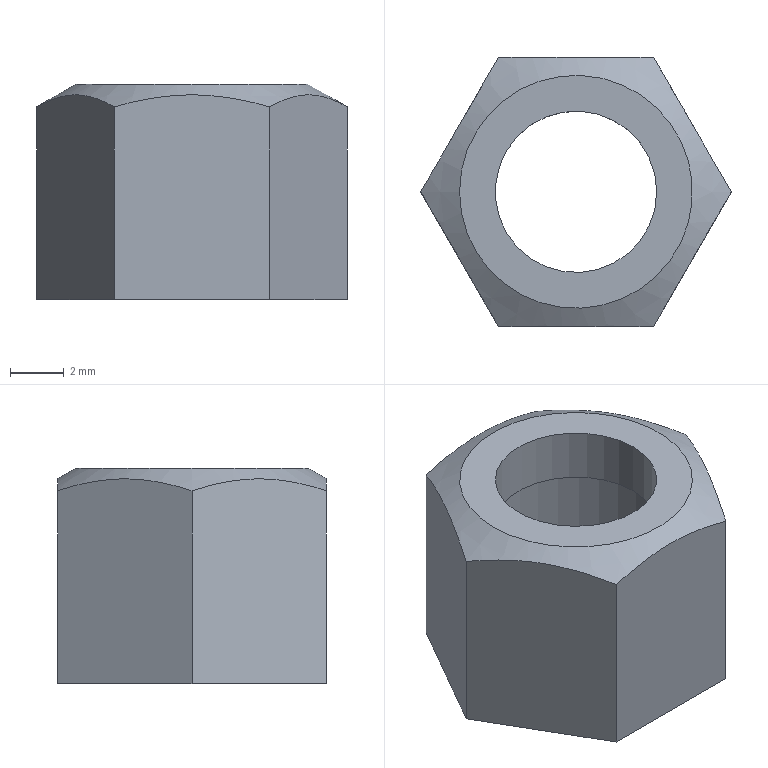Component | NX | PIPE_CAP_3 | 1 solid | 12 faces | box 11.55 x 10 x 8 mm | volume 327 mm3 | plane 9 | cylinder 2 | cone 1 | commonest cylinder face diameters 8 x1 6 x1
STEP:
#1=CARTESIAN_POINT('',(0.,0.,0.));
#2=DIRECTION('',(0.,0.,1.));
#3=DIRECTION('',(1.,0.,0.));
#4=AXIS2_PLACEMENT_3D('',#1,#2,#3);
#5=CARTESIAN_POINT('',(-105.726,59.,47.667));
#6=VERTEX_POINT('',#5);
#7=CARTESIAN_POINT('',(-105.726,59.,40.5));
#8=VERTEX_POINT('',#7);
#9=CARTESIAN_POINT('',(-105.726,59.,48.5));
#10=DIRECTION('',(0.,0.,-1.));
#11=VECTOR('',#10,1.);
#12=LINE('',#9,#11);
#13=CARTESIAN_POINT('',(-108.613,54.,48.5));
#14=DIRECTION('',(-0.866,0.5,0.));
#15=DIRECTION('',(-0.5,-0.866,0.));
#16=AXIS2_PLACEMENT_3D('',#13,#14,#15);
#17=PLANE('',#16);
#18=CARTESIAN_POINT('',(-5.774,0.));
#19=DIRECTION('',(0.,-1.));
#20=VECTOR('',#19,1.);
#21=LINE('',#18,#20);
#22=(GEOMETRIC_REPRESENTATION_CONTEXT(2)PARAMETRIC_REPRESENTATION_CONTEXT()REPRESENTATION_CONTEXT('',''));
#23=DEFINITIONAL_REPRESENTATION('',(#21),#22);
#24=PCURVE('',#17,#23);
#25=CARTESIAN_POINT('',(-105.726,59.,48.5));
#26=DIRECTION('',(-0.866,-0.5,0.));
#27=DIRECTION('',(0.5,-0.866,0.));
#28=AXIS2_PLACEMENT_3D('',#25,#26,#27);
#29=PLANE('',#28);
#30=CARTESIAN_POINT('',(0.,0.));
#31=DIRECTION('',(0.,-1.));
#32=VECTOR('',#31,1.);
#33=LINE('',#30,#32);
#34=(GEOMETRIC_REPRESENTATION_CONTEXT(2)PARAMETRIC_REPRESENTATION_CONTEXT()REPRESENTATION_CONTEXT('',''));
#35=DEFINITIONAL_REPRESENTATION('',(#33),#34);
#36=PCURVE('',#29,#35);
#37=SURFACE_CURVE('',#12,(#24,#36),.PCURVE_S1.);
#38=EDGE_CURVE('',#6,#8,#37,.T.);
#39=ORIENTED_EDGE('',*,*,#38,.F.);
#40=CARTESIAN_POINT('',(-108.613,54.,47.667));
#41=VERTEX_POINT('',#40);
#42=CARTESIAN_POINT('',(-105.726,59.,47.667));
#43=CARTESIAN_POINT('',(-106.198,58.184,47.939));
#44=CARTESIAN_POINT('',(-106.676,57.355,48.113));
#45=CARTESIAN_POINT('',(-107.658,55.655,48.114));
#46=CARTESIAN_POINT('',(-108.141,54.817,47.939));
#47=CARTESIAN_POINT('',(-108.613,54.,47.667));
#48=B_SPLINE_CURVE_WITH_KNOTS('',3,(#42,#43,#44,#45,#46,#47),.UNSPECIFIED.,.F.,.F.,(4,2,4),(0.,0.5,1.),.UNSPECIFIED.);
#49=CARTESIAN_POINT('',(-5.774,-0.8333));
#50=CARTESIAN_POINT('',(-4.831,-0.5612));
#51=CARTESIAN_POINT('',(-3.874,-0.3874));
#52=CARTESIAN_POINT('',(-1.911,-0.3861));
#53=CARTESIAN_POINT('',(-0.9439,-0.5609));
#54=CARTESIAN_POINT('',(0.,-0.8333));
#55=B_SPLINE_CURVE_WITH_KNOTS('',3,(#49,#50,#51,#52,#53,#54),.UNSPECIFIED.,.F.,.F.,(4,2,4),(0.,0.5,1.),.UNSPECIFIED.);
#56=(GEOMETRIC_REPRESENTATION_CONTEXT(2)PARAMETRIC_REPRESENTATION_CONTEXT()REPRESENTATION_CONTEXT('',''));
#57=DEFINITIONAL_REPRESENTATION('',(#55),#56);
#58=PCURVE('',#17,#57);
#59=CARTESIAN_POINT('',(-111.5,59.,48.5));
#60=DIRECTION('',(0.,0.,-1.));
#61=DIRECTION('',(-1.,0.,0.));
#62=AXIS2_PLACEMENT_3D('',#59,#60,#61);
#63=CONICAL_SURFACE('',#62,4.33,1.047);
#64=CARTESIAN_POINT('',(3.142,0.8333));
#65=CARTESIAN_POINT('',(3.154,0.8086));
#66=CARTESIAN_POINT('',(3.181,0.7607));
#67=CARTESIAN_POINT('',(3.222,0.694));
#68=CARTESIAN_POINT('',(3.265,0.6329));
#69=CARTESIAN_POINT('',(3.31,0.5776));
#70=CARTESIAN_POINT('',(3.357,0.5285));
#71=CARTESIAN_POINT('',(3.405,0.4861));
#72=CARTESIAN_POINT('',(3.455,0.4507));
#73=CARTESIAN_POINT('',(3.506,0.4227));
#74=CARTESIAN_POINT('',(3.558,0.4022));
#75=CARTESIAN_POINT('',(3.611,0.3897));
#76=CARTESIAN_POINT('',(3.664,0.3854));
#77=CARTESIAN_POINT('',(3.718,0.3894));
#78=CARTESIAN_POINT('',(3.771,0.4016));
#79=CARTESIAN_POINT('',(3.823,0.4219));
#80=CARTESIAN_POINT('',(3.874,0.4498));
#81=CARTESIAN_POINT('',(3.924,0.4852));
#82=CARTESIAN_POINT('',(3.973,0.5277));
#83=CARTESIAN_POINT('',(4.02,0.5769));
#84=CARTESIAN_POINT('',(4.065,0.6323));
#85=CARTESIAN_POINT('',(4.108,0.6937));
#86=CARTESIAN_POINT('',(4.15,0.7606));
#87=CARTESIAN_POINT('',(4.176,0.8086));
#88=CARTESIAN_POINT('',(4.189,0.8333));
#89=B_SPLINE_CURVE_WITH_KNOTS('',3,(#64,#65,#66,#67,#68,#69,#70,#71,#72,#73,#74,#75,#76,#77,#78,#79,#80,#81,#82,#83,#84,#85,#86,#87,#88),.UNSPECIFIED.,.F.,.F.,(4,1,1,1,1,1,1,1,1,1,1,1,1,1,1,1,1,1,1,1,1,1,4),(0.,0.04545,0.09091,0.1364,0.1818,0.2273,0.2727,0.3182,0.3636,0.4091,0.4545,0.5,0.5455,0.5909,0.6364,0.6818,0.7273,0.7727,0.8182,0.8636,0.9091,0.9545,1.),.QUASI_UNIFORM_KNOTS.);
#90=(GEOMETRIC_REPRESENTATION_CONTEXT(2)PARAMETRIC_REPRESENTATION_CONTEXT()REPRESENTATION_CONTEXT('',''));
#91=DEFINITIONAL_REPRESENTATION('',(#89),#90);
#92=PCURVE('',#63,#91);
#93=SURFACE_CURVE('',#48,(#58,#92),.PCURVE_S1.);
#94=EDGE_CURVE('',#6,#41,#93,.T.);
#95=ORIENTED_EDGE('',*,*,#94,.T.);
#96=CARTESIAN_POINT('',(-108.613,54.,40.5));
#97=VERTEX_POINT('',#96);
#98=CARTESIAN_POINT('',(-108.613,54.,48.5));
#99=DIRECTION('',(0.,0.,-1.));
#100=VECTOR('',#99,1.);
#101=LINE('',#98,#100);
#102=CARTESIAN_POINT('',(0.,0.));
#103=DIRECTION('',(0.,-1.));
#104=VECTOR('',#103,1.);
#105=LINE('',#102,#104);
#106=(GEOMETRIC_REPRESENTATION_CONTEXT(2)PARAMETRIC_REPRESENTATION_CONTEXT()REPRESENTATION_CONTEXT('',''));
#107=DEFINITIONAL_REPRESENTATION('',(#105),#106);
#108=PCURVE('',#17,#107);
#109=CARTESIAN_POINT('',(-114.387,54.,48.5));
#110=DIRECTION('',(0.,1.,0.));
#111=DIRECTION('',(-1.,0.,0.));
#112=AXIS2_PLACEMENT_3D('',#109,#110,#111);
#113=PLANE('',#112);
#114=CARTESIAN_POINT('',(-5.774,0.));
#115=DIRECTION('',(0.,-1.));
#116=VECTOR('',#115,1.);
#117=LINE('',#114,#116);
#118=(GEOMETRIC_REPRESENTATION_CONTEXT(2)PARAMETRIC_REPRESENTATION_CONTEXT()REPRESENTATION_CONTEXT('',''));
#119=DEFINITIONAL_REPRESENTATION('',(#117),#118);
#120=PCURVE('',#113,#119);
#121=SURFACE_CURVE('',#101,(#108,#120),.PCURVE_S1.);
#122=EDGE_CURVE('',#41,#97,#121,.T.);
#123=ORIENTED_EDGE('',*,*,#122,.T.);
#124=CARTESIAN_POINT('',(-108.613,54.,40.5));
#125=DIRECTION('',(0.5,0.866,0.));
#126=VECTOR('',#125,1.);
#127=LINE('',#124,#126);
#128=CARTESIAN_POINT('',(0.,-8.));
#129=DIRECTION('',(-1.,0.));
#130=VECTOR('',#129,1.);
#131=LINE('',#128,#130);
#132=(GEOMETRIC_REPRESENTATION_CONTEXT(2)PARAMETRIC_REPRESENTATION_CONTEXT()REPRESENTATION_CONTEXT('',''));
#133=DEFINITIONAL_REPRESENTATION('',(#131),#132);
#134=PCURVE('',#17,#133);
#135=CARTESIAN_POINT('',(-111.5,59.,40.5));
#136=DIRECTION('',(0.,0.,1.));
#137=DIRECTION('',(1.,0.,0.));
#138=AXIS2_PLACEMENT_3D('',#135,#136,#137);
#139=PLANE('',#138);
#140=CARTESIAN_POINT('',(2.887,-5.));
#141=DIRECTION('',(0.5,0.866));
#142=VECTOR('',#141,1.);
#143=LINE('',#140,#142);
#144=(GEOMETRIC_REPRESENTATION_CONTEXT(2)PARAMETRIC_REPRESENTATION_CONTEXT()REPRESENTATION_CONTEXT('',''));
#145=DEFINITIONAL_REPRESENTATION('',(#143),#144);
#146=PCURVE('',#139,#145);
#147=SURFACE_CURVE('',#127,(#134,#146),.PCURVE_S1.);
#148=EDGE_CURVE('',#97,#8,#147,.T.);
#149=ORIENTED_EDGE('',*,*,#148,.T.);
#150=EDGE_LOOP('',(#39,#95,#123,#149));
#151=FACE_BOUND('',#150,.T.);
#152=ADVANCED_FACE('',(#151),#17,.F.);
#153=CARTESIAN_POINT('',(-108.613,64.,47.667));
#154=VERTEX_POINT('',#153);
#155=CARTESIAN_POINT('',(-108.613,64.,40.5));
#156=VERTEX_POINT('',#155);
#157=CARTESIAN_POINT('',(-108.613,64.,48.5));
#158=DIRECTION('',(0.,0.,-1.));
#159=VECTOR('',#158,1.);
#160=LINE('',#157,#159);
#161=CARTESIAN_POINT('',(-5.774,0.));
#162=DIRECTION('',(0.,-1.));
#163=VECTOR('',#162,1.);
#164=LINE('',#161,#163);
#165=(GEOMETRIC_REPRESENTATION_CONTEXT(2)PARAMETRIC_REPRESENTATION_CONTEXT()REPRESENTATION_CONTEXT('',''));
#166=DEFINITIONAL_REPRESENTATION('',(#164),#165);
#167=PCURVE('',#29,#166);
#168=CARTESIAN_POINT('',(-108.613,64.,48.5));
#169=DIRECTION('',(0.,-1.,0.));
#170=DIRECTION('',(1.,0.,0.));
#171=AXIS2_PLACEMENT_3D('',#168,#169,#170);
#172=PLANE('',#171);
#173=CARTESIAN_POINT('',(0.,0.));
#174=DIRECTION('',(0.,-1.));
#175=VECTOR('',#174,1.);
#176=LINE('',#173,#175);
#177=(GEOMETRIC_REPRESENTATION_CONTEXT(2)PARAMETRIC_REPRESENTATION_CONTEXT()REPRESENTATION_CONTEXT('',''));
#178=DEFINITIONAL_REPRESENTATION('',(#176),#177);
#179=PCURVE('',#172,#178);
#180=SURFACE_CURVE('',#160,(#167,#179),.PCURVE_S1.);
#181=EDGE_CURVE('',#154,#156,#180,.T.);
#182=ORIENTED_EDGE('',*,*,#181,.F.);
#183=CARTESIAN_POINT('',(-108.613,64.,47.667));
#184=CARTESIAN_POINT('',(-108.142,63.184,47.939));
#185=CARTESIAN_POINT('',(-107.663,62.355,48.113));
#186=CARTESIAN_POINT('',(-106.682,60.655,48.114));
#187=CARTESIAN_POINT('',(-106.198,59.817,47.939));
#188=CARTESIAN_POINT('',(-105.726,59.,47.667));
#189=B_SPLINE_CURVE_WITH_KNOTS('',3,(#183,#184,#185,#186,#187,#188),.UNSPECIFIED.,.F.,.F.,(4,2,4),(0.,0.5,1.),.UNSPECIFIED.);
#190=CARTESIAN_POINT('',(-5.774,-0.8333));
#191=CARTESIAN_POINT('',(-4.831,-0.5612));
#192=CARTESIAN_POINT('',(-3.874,-0.3874));
#193=CARTESIAN_POINT('',(-1.911,-0.3861));
#194=CARTESIAN_POINT('',(-0.9439,-0.5609));
#195=CARTESIAN_POINT('',(0.,-0.8333));
#196=B_SPLINE_CURVE_WITH_KNOTS('',3,(#190,#191,#192,#193,#194,#195),.UNSPECIFIED.,.F.,.F.,(4,2,4),(0.,0.5,1.),.UNSPECIFIED.);
#197=(GEOMETRIC_REPRESENTATION_CONTEXT(2)PARAMETRIC_REPRESENTATION_CONTEXT()REPRESENTATION_CONTEXT('',''));
#198=DEFINITIONAL_REPRESENTATION('',(#196),#197);
#199=PCURVE('',#29,#198);
#200=CARTESIAN_POINT('',(2.094,0.8333));
#201=CARTESIAN_POINT('',(2.107,0.8086));
#202=CARTESIAN_POINT('',(2.134,0.7607));
#203=CARTESIAN_POINT('',(2.175,0.694));
#204=CARTESIAN_POINT('',(2.218,0.6329));
#205=CARTESIAN_POINT('',(2.263,0.5776));
#206=CARTESIAN_POINT('',(2.31,0.5285));
#207=CARTESIAN_POINT('',(2.358,0.4861));
#208=CARTESIAN_POINT('',(2.408,0.4507));
#209=CARTESIAN_POINT('',(2.458,0.4227));
#210=CARTESIAN_POINT('',(2.511,0.4022));
#211=CARTESIAN_POINT('',(2.563,0.3897));
#212=CARTESIAN_POINT('',(2.617,0.3854));
#213=CARTESIAN_POINT('',(2.67,0.3894));
#214=CARTESIAN_POINT('',(2.723,0.4016));
#215=CARTESIAN_POINT('',(2.776,0.4219));
#216=CARTESIAN_POINT('',(2.827,0.4498));
#217=CARTESIAN_POINT('',(2.877,0.4852));
#218=CARTESIAN_POINT('',(2.925,0.5277));
#219=CARTESIAN_POINT('',(2.972,0.5769));
#220=CARTESIAN_POINT('',(3.018,0.6323));
#221=CARTESIAN_POINT('',(3.061,0.6937));
#222=CARTESIAN_POINT('',(3.102,0.7606));
#223=CARTESIAN_POINT('',(3.129,0.8086));
#224=CARTESIAN_POINT('',(3.142,0.8333));
#225=B_SPLINE_CURVE_WITH_KNOTS('',3,(#200,#201,#202,#203,#204,#205,#206,#207,#208,#209,#210,#211,#212,#213,#214,#215,#216,#217,#218,#219,#220,#221,#222,#223,#224),.UNSPECIFIED.,.F.,.F.,(4,1,1,1,1,1,1,1,1,1,1,1,1,1,1,1,1,1,1,1,1,1,4),(0.,0.04545,0.09091,0.1364,0.1818,0.2273,0.2727,0.3182,0.3636,0.4091,0.4545,0.5,0.5455,0.5909,0.6364,0.6818,0.7273,0.7727,0.8182,0.8636,0.9091,0.9545,1.),.QUASI_UNIFORM_KNOTS.);
#226=(GEOMETRIC_REPRESENTATION_CONTEXT(2)PARAMETRIC_REPRESENTATION_CONTEXT()REPRESENTATION_CONTEXT('',''));
#227=DEFINITIONAL_REPRESENTATION('',(#225),#226);
#228=PCURVE('',#63,#227);
#229=SURFACE_CURVE('',#189,(#199,#228),.PCURVE_S1.);
#230=EDGE_CURVE('',#154,#6,#229,.T.);
#231=ORIENTED_EDGE('',*,*,#230,.T.);
#232=ORIENTED_EDGE('',*,*,#38,.T.);
#233=CARTESIAN_POINT('',(-105.726,59.,40.5));
#234=DIRECTION('',(-0.5,0.866,0.));
#235=VECTOR('',#234,1.);
#236=LINE('',#233,#235);
#237=CARTESIAN_POINT('',(0.,-8.));
#238=DIRECTION('',(-1.,0.));
#239=VECTOR('',#238,1.);
#240=LINE('',#237,#239);
#241=(GEOMETRIC_REPRESENTATION_CONTEXT(2)PARAMETRIC_REPRESENTATION_CONTEXT()REPRESENTATION_CONTEXT('',''));
#242=DEFINITIONAL_REPRESENTATION('',(#240),#241);
#243=PCURVE('',#29,#242);
#244=CARTESIAN_POINT('',(5.774,-0.));
#245=DIRECTION('',(-0.5,0.866));
#246=VECTOR('',#245,1.);
#247=LINE('',#244,#246);
#248=(GEOMETRIC_REPRESENTATION_CONTEXT(2)PARAMETRIC_REPRESENTATION_CONTEXT()REPRESENTATION_CONTEXT('',''));
#249=DEFINITIONAL_REPRESENTATION('',(#247),#248);
#250=PCURVE('',#139,#249);
#251=SURFACE_CURVE('',#236,(#243,#250),.PCURVE_S1.);
#252=EDGE_CURVE('',#8,#156,#251,.T.);
#253=ORIENTED_EDGE('',*,*,#252,.T.);
#254=EDGE_LOOP('',(#182,#231,#232,#253));
#255=FACE_BOUND('',#254,.T.);
#256=ADVANCED_FACE('',(#255),#29,.F.);
#257=CARTESIAN_POINT('',(-114.387,64.,47.667));
#258=VERTEX_POINT('',#257);
#259=CARTESIAN_POINT('',(-114.387,64.,40.5));
#260=VERTEX_POINT('',#259);
#261=CARTESIAN_POINT('',(-114.387,64.,48.5));
#262=DIRECTION('',(0.,0.,-1.));
#263=VECTOR('',#262,1.);
#264=LINE('',#261,#263);
#265=CARTESIAN_POINT('',(-5.774,0.));
#266=DIRECTION('',(0.,-1.));
#267=VECTOR('',#266,1.);
#268=LINE('',#265,#267);
#269=(GEOMETRIC_REPRESENTATION_CONTEXT(2)PARAMETRIC_REPRESENTATION_CONTEXT()REPRESENTATION_CONTEXT('',''));
#270=DEFINITIONAL_REPRESENTATION('',(#268),#269);
#271=PCURVE('',#172,#270);
#272=CARTESIAN_POINT('',(-114.387,64.,48.5));
#273=DIRECTION('',(0.866,-0.5,0.));
#274=DIRECTION('',(0.5,0.866,0.));
#275=AXIS2_PLACEMENT_3D('',#272,#273,#274);
#276=PLANE('',#275);
#277=CARTESIAN_POINT('',(0.,0.));
#278=DIRECTION('',(0.,-1.));
#279=VECTOR('',#278,1.);
#280=LINE('',#277,#279);
#281=(GEOMETRIC_REPRESENTATION_CONTEXT(2)PARAMETRIC_REPRESENTATION_CONTEXT()REPRESENTATION_CONTEXT('',''));
#282=DEFINITIONAL_REPRESENTATION('',(#280),#281);
#283=PCURVE('',#276,#282);
#284=SURFACE_CURVE('',#264,(#271,#283),.PCURVE_S1.);
#285=EDGE_CURVE('',#258,#260,#284,.T.);
#286=ORIENTED_EDGE('',*,*,#285,.F.);
#287=CARTESIAN_POINT('',(-114.387,64.,47.667));
#288=CARTESIAN_POINT('',(-113.448,64.,47.938));
#289=CARTESIAN_POINT('',(-112.475,64.,48.113));
#290=CARTESIAN_POINT('',(-110.524,64.,48.113));
#291=CARTESIAN_POINT('',(-109.546,64.,47.936));
#292=CARTESIAN_POINT('',(-108.613,64.,47.667));
#293=B_SPLINE_CURVE_WITH_KNOTS('',3,(#287,#288,#289,#290,#291,#292),.UNSPECIFIED.,.F.,.F.,(4,2,4),(0.,0.5,1.),.UNSPECIFIED.);
#294=CARTESIAN_POINT('',(-5.774,-0.8333));
#295=CARTESIAN_POINT('',(-4.835,-0.5623));
#296=CARTESIAN_POINT('',(-3.862,-0.3867));
#297=CARTESIAN_POINT('',(-1.91,-0.3868));
#298=CARTESIAN_POINT('',(-0.9332,-0.5639));
#299=CARTESIAN_POINT('',(0.,-0.8333));
#300=B_SPLINE_CURVE_WITH_KNOTS('',3,(#294,#295,#296,#297,#298,#299),.UNSPECIFIED.,.F.,.F.,(4,2,4),(0.,0.5,1.),.UNSPECIFIED.);
#301=(GEOMETRIC_REPRESENTATION_CONTEXT(2)PARAMETRIC_REPRESENTATION_CONTEXT()REPRESENTATION_CONTEXT('',''));
#302=DEFINITIONAL_REPRESENTATION('',(#300),#301);
#303=PCURVE('',#172,#302);
#304=CARTESIAN_POINT('',(1.047,0.8333));
#305=CARTESIAN_POINT('',(1.06,0.8087));
#306=CARTESIAN_POINT('',(1.086,0.7609));
#307=CARTESIAN_POINT('',(1.128,0.6942));
#308=CARTESIAN_POINT('',(1.171,0.6329));
#309=CARTESIAN_POINT('',(1.216,0.5774));
#310=CARTESIAN_POINT('',(1.263,0.5282));
#311=CARTESIAN_POINT('',(1.312,0.4856));
#312=CARTESIAN_POINT('',(1.362,0.4502));
#313=CARTESIAN_POINT('',(1.413,0.4221));
#314=CARTESIAN_POINT('',(1.465,0.4018));
#315=CARTESIAN_POINT('',(1.518,0.3895));
#316=CARTESIAN_POINT('',(1.571,0.3854));
#317=CARTESIAN_POINT('',(1.624,0.3896));
#318=CARTESIAN_POINT('',(1.677,0.4019));
#319=CARTESIAN_POINT('',(1.729,0.4224));
#320=CARTESIAN_POINT('',(1.781,0.4505));
#321=CARTESIAN_POINT('',(1.831,0.4861));
#322=CARTESIAN_POINT('',(1.879,0.5287));
#323=CARTESIAN_POINT('',(1.926,0.578));
#324=CARTESIAN_POINT('',(1.971,0.6335));
#325=CARTESIAN_POINT('',(2.014,0.6948));
#326=CARTESIAN_POINT('',(2.056,0.7613));
#327=CARTESIAN_POINT('',(2.082,0.8088));
#328=CARTESIAN_POINT('',(2.094,0.8333));
#329=B_SPLINE_CURVE_WITH_KNOTS('',3,(#304,#305,#306,#307,#308,#309,#310,#311,#312,#313,#314,#315,#316,#317,#318,#319,#320,#321,#322,#323,#324,#325,#326,#327,#328),.UNSPECIFIED.,.F.,.F.,(4,1,1,1,1,1,1,1,1,1,1,1,1,1,1,1,1,1,1,1,1,1,4),(0.,0.04545,0.09091,0.1364,0.1818,0.2273,0.2727,0.3182,0.3636,0.4091,0.4545,0.5,0.5455,0.5909,0.6364,0.6818,0.7273,0.7727,0.8182,0.8636,0.9091,0.9545,1.),.QUASI_UNIFORM_KNOTS.);
#330=(GEOMETRIC_REPRESENTATION_CONTEXT(2)PARAMETRIC_REPRESENTATION_CONTEXT()REPRESENTATION_CONTEXT('',''));
#331=DEFINITIONAL_REPRESENTATION('',(#329),#330);
#332=PCURVE('',#63,#331);
#333=SURFACE_CURVE('',#293,(#303,#332),.PCURVE_S1.);
#334=EDGE_CURVE('',#258,#154,#333,.T.);
#335=ORIENTED_EDGE('',*,*,#334,.T.);
#336=ORIENTED_EDGE('',*,*,#181,.T.);
#337=CARTESIAN_POINT('',(-108.613,64.,40.5));
#338=DIRECTION('',(-1.,-0.,0.));
#339=VECTOR('',#338,1.);
#340=LINE('',#337,#339);
#341=CARTESIAN_POINT('',(0.,-8.));
#342=DIRECTION('',(-1.,0.));
#343=VECTOR('',#342,1.);
#344=LINE('',#341,#343);
#345=(GEOMETRIC_REPRESENTATION_CONTEXT(2)PARAMETRIC_REPRESENTATION_CONTEXT()REPRESENTATION_CONTEXT('',''));
#346=DEFINITIONAL_REPRESENTATION('',(#344),#345);
#347=PCURVE('',#172,#346);
#348=CARTESIAN_POINT('',(2.887,5.));
#349=DIRECTION('',(-1.,-0.));
#350=VECTOR('',#349,1.);
#351=LINE('',#348,#350);
#352=(GEOMETRIC_REPRESENTATION_CONTEXT(2)PARAMETRIC_REPRESENTATION_CONTEXT()REPRESENTATION_CONTEXT('',''));
#353=DEFINITIONAL_REPRESENTATION('',(#351),#352);
#354=PCURVE('',#139,#353);
#355=SURFACE_CURVE('',#340,(#347,#354),.PCURVE_S1.);
#356=EDGE_CURVE('',#156,#260,#355,.T.);
#357=ORIENTED_EDGE('',*,*,#356,.T.);
#358=EDGE_LOOP('',(#286,#335,#336,#357));
#359=FACE_BOUND('',#358,.T.);
#360=ADVANCED_FACE('',(#359),#172,.F.);
#361=CARTESIAN_POINT('',(-117.274,59.,47.667));
#362=VERTEX_POINT('',#361);
#363=CARTESIAN_POINT('',(-117.274,59.,40.5));
#364=VERTEX_POINT('',#363);
#365=CARTESIAN_POINT('',(-117.274,59.,48.5));
#366=DIRECTION('',(0.,0.,-1.));
#367=VECTOR('',#366,1.);
#368=LINE('',#365,#367);
#369=CARTESIAN_POINT('',(-5.774,0.));
#370=DIRECTION('',(0.,-1.));
#371=VECTOR('',#370,1.);
#372=LINE('',#369,#371);
#373=(GEOMETRIC_REPRESENTATION_CONTEXT(2)PARAMETRIC_REPRESENTATION_CONTEXT()REPRESENTATION_CONTEXT('',''));
#374=DEFINITIONAL_REPRESENTATION('',(#372),#373);
#375=PCURVE('',#276,#374);
#376=CARTESIAN_POINT('',(-117.274,59.,48.5));
#377=DIRECTION('',(0.866,0.5,0.));
#378=DIRECTION('',(-0.5,0.866,0.));
#379=AXIS2_PLACEMENT_3D('',#376,#377,#378);
#380=PLANE('',#379);
#381=CARTESIAN_POINT('',(0.,0.));
#382=DIRECTION('',(0.,-1.));
#383=VECTOR('',#382,1.);
#384=LINE('',#381,#383);
#385=(GEOMETRIC_REPRESENTATION_CONTEXT(2)PARAMETRIC_REPRESENTATION_CONTEXT()REPRESENTATION_CONTEXT('',''));
#386=DEFINITIONAL_REPRESENTATION('',(#384),#385);
#387=PCURVE('',#380,#386);
#388=SURFACE_CURVE('',#368,(#375,#387),.PCURVE_S1.);
#389=EDGE_CURVE('',#362,#364,#388,.T.);
#390=ORIENTED_EDGE('',*,*,#389,.F.);
#391=CARTESIAN_POINT('',(-117.274,59.,47.667));
#392=CARTESIAN_POINT('',(-116.802,59.816,47.939));
#393=CARTESIAN_POINT('',(-116.324,60.645,48.113));
#394=CARTESIAN_POINT('',(-115.342,62.345,48.114));
#395=CARTESIAN_POINT('',(-114.859,63.183,47.939));
#396=CARTESIAN_POINT('',(-114.387,64.,47.667));
#397=B_SPLINE_CURVE_WITH_KNOTS('',3,(#391,#392,#393,#394,#395,#396),.UNSPECIFIED.,.F.,.F.,(4,2,4),(0.,0.5,1.),.UNSPECIFIED.);
#398=CARTESIAN_POINT('',(-5.774,-0.8333));
#399=CARTESIAN_POINT('',(-4.831,-0.5612));
#400=CARTESIAN_POINT('',(-3.874,-0.3874));
#401=CARTESIAN_POINT('',(-1.911,-0.3861));
#402=CARTESIAN_POINT('',(-0.9439,-0.5609));
#403=CARTESIAN_POINT('',(0.,-0.8333));
#404=B_SPLINE_CURVE_WITH_KNOTS('',3,(#398,#399,#400,#401,#402,#403),.UNSPECIFIED.,.F.,.F.,(4,2,4),(0.,0.5,1.),.UNSPECIFIED.);
#405=(GEOMETRIC_REPRESENTATION_CONTEXT(2)PARAMETRIC_REPRESENTATION_CONTEXT()REPRESENTATION_CONTEXT('',''));
#406=DEFINITIONAL_REPRESENTATION('',(#404),#405);
#407=PCURVE('',#276,#406);
#408=CARTESIAN_POINT('',(0.,0.8333));
#409=CARTESIAN_POINT('',(0.01285,0.8086));
#410=CARTESIAN_POINT('',(0.03917,0.7607));
#411=CARTESIAN_POINT('',(0.08049,0.694));
#412=CARTESIAN_POINT('',(0.1236,0.6329));
#413=CARTESIAN_POINT('',(0.1685,0.5776));
#414=CARTESIAN_POINT('',(0.2152,0.5285));
#415=CARTESIAN_POINT('',(0.2634,0.4861));
#416=CARTESIAN_POINT('',(0.3131,0.4507));
#417=CARTESIAN_POINT('',(0.3641,0.4227));
#418=CARTESIAN_POINT('',(0.4162,0.4022));
#419=CARTESIAN_POINT('',(0.469,0.3897));
#420=CARTESIAN_POINT('',(0.5225,0.3854));
#421=CARTESIAN_POINT('',(0.576,0.3894));
#422=CARTESIAN_POINT('',(0.629,0.4016));
#423=CARTESIAN_POINT('',(0.6813,0.4219));
#424=CARTESIAN_POINT('',(0.7325,0.4498));
#425=CARTESIAN_POINT('',(0.7825,0.4852));
#426=CARTESIAN_POINT('',(0.8311,0.5277));
#427=CARTESIAN_POINT('',(0.878,0.5769));
#428=CARTESIAN_POINT('',(0.9232,0.6323));
#429=CARTESIAN_POINT('',(0.9665,0.6937));
#430=CARTESIAN_POINT('',(1.008,0.7606));
#431=CARTESIAN_POINT('',(1.034,0.8086));
#432=CARTESIAN_POINT('',(1.047,0.8333));
#433=B_SPLINE_CURVE_WITH_KNOTS('',3,(#408,#409,#410,#411,#412,#413,#414,#415,#416,#417,#418,#419,#420,#421,#422,#423,#424,#425,#426,#427,#428,#429,#430,#431,#432),.UNSPECIFIED.,.F.,.F.,(4,1,1,1,1,1,1,1,1,1,1,1,1,1,1,1,1,1,1,1,1,1,4),(0.,0.04545,0.09091,0.1364,0.1818,0.2273,0.2727,0.3182,0.3636,0.4091,0.4545,0.5,0.5455,0.5909,0.6364,0.6818,0.7273,0.7727,0.8182,0.8636,0.9091,0.9545,1.),.QUASI_UNIFORM_KNOTS.);
#434=(GEOMETRIC_REPRESENTATION_CONTEXT(2)PARAMETRIC_REPRESENTATION_CONTEXT()REPRESENTATION_CONTEXT('',''));
#435=DEFINITIONAL_REPRESENTATION('',(#433),#434);
#436=PCURVE('',#63,#435);
#437=SURFACE_CURVE('',#397,(#407,#436),.PCURVE_S1.);
#438=EDGE_CURVE('',#362,#258,#437,.T.);
#439=ORIENTED_EDGE('',*,*,#438,.T.);
#440=ORIENTED_EDGE('',*,*,#285,.T.);
#441=CARTESIAN_POINT('',(-114.387,64.,40.5));
#442=DIRECTION('',(-0.5,-0.866,0.));
#443=VECTOR('',#442,1.);
#444=LINE('',#441,#443);
#445=CARTESIAN_POINT('',(0.,-8.));
#446=DIRECTION('',(-1.,0.));
#447=VECTOR('',#446,1.);
#448=LINE('',#445,#447);
#449=(GEOMETRIC_REPRESENTATION_CONTEXT(2)PARAMETRIC_REPRESENTATION_CONTEXT()REPRESENTATION_CONTEXT('',''));
#450=DEFINITIONAL_REPRESENTATION('',(#448),#449);
#451=PCURVE('',#276,#450);
#452=CARTESIAN_POINT('',(-2.887,5.));
#453=DIRECTION('',(-0.5,-0.866));
#454=VECTOR('',#453,1.);
#455=LINE('',#452,#454);
#456=(GEOMETRIC_REPRESENTATION_CONTEXT(2)PARAMETRIC_REPRESENTATION_CONTEXT()REPRESENTATION_CONTEXT('',''));
#457=DEFINITIONAL_REPRESENTATION('',(#455),#456);
#458=PCURVE('',#139,#457);
#459=SURFACE_CURVE('',#444,(#451,#458),.PCURVE_S1.);
#460=EDGE_CURVE('',#260,#364,#459,.T.);
#461=ORIENTED_EDGE('',*,*,#460,.T.);
#462=EDGE_LOOP('',(#390,#439,#440,#461));
#463=FACE_BOUND('',#462,.T.);
#464=ADVANCED_FACE('',(#463),#276,.F.);
#465=CARTESIAN_POINT('',(-114.387,54.,47.667));
#466=VERTEX_POINT('',#465);
#467=CARTESIAN_POINT('',(-114.387,54.,40.5));
#468=VERTEX_POINT('',#467);
#469=CARTESIAN_POINT('',(-114.387,54.,48.5));
#470=DIRECTION('',(0.,0.,-1.));
#471=VECTOR('',#470,1.);
#472=LINE('',#469,#471);
#473=CARTESIAN_POINT('',(-5.774,0.));
#474=DIRECTION('',(0.,-1.));
#475=VECTOR('',#474,1.);
#476=LINE('',#473,#475);
#477=(GEOMETRIC_REPRESENTATION_CONTEXT(2)PARAMETRIC_REPRESENTATION_CONTEXT()REPRESENTATION_CONTEXT('',''));
#478=DEFINITIONAL_REPRESENTATION('',(#476),#477);
#479=PCURVE('',#380,#478);
#480=CARTESIAN_POINT('',(0.,0.));
#481=DIRECTION('',(0.,-1.));
#482=VECTOR('',#481,1.);
#483=LINE('',#480,#482);
#484=(GEOMETRIC_REPRESENTATION_CONTEXT(2)PARAMETRIC_REPRESENTATION_CONTEXT()REPRESENTATION_CONTEXT('',''));
#485=DEFINITIONAL_REPRESENTATION('',(#483),#484);
#486=PCURVE('',#113,#485);
#487=SURFACE_CURVE('',#472,(#479,#486),.PCURVE_S1.);
#488=EDGE_CURVE('',#466,#468,#487,.T.);
#489=ORIENTED_EDGE('',*,*,#488,.F.);
#490=CARTESIAN_POINT('',(-114.387,54.,47.667));
#491=CARTESIAN_POINT('',(-114.858,54.816,47.939));
#492=CARTESIAN_POINT('',(-115.337,55.645,48.113));
#493=CARTESIAN_POINT('',(-116.318,57.345,48.114));
#494=CARTESIAN_POINT('',(-116.802,58.183,47.939));
#495=CARTESIAN_POINT('',(-117.274,59.,47.667));
#496=B_SPLINE_CURVE_WITH_KNOTS('',3,(#490,#491,#492,#493,#494,#495),.UNSPECIFIED.,.F.,.F.,(4,2,4),(0.,0.5,1.),.UNSPECIFIED.);
#497=CARTESIAN_POINT('',(-5.774,-0.8333));
#498=CARTESIAN_POINT('',(-4.831,-0.5612));
#499=CARTESIAN_POINT('',(-3.874,-0.3874));
#500=CARTESIAN_POINT('',(-1.911,-0.3861));
#501=CARTESIAN_POINT('',(-0.9439,-0.5609));
#502=CARTESIAN_POINT('',(0.,-0.8333));
#503=B_SPLINE_CURVE_WITH_KNOTS('',3,(#497,#498,#499,#500,#501,#502),.UNSPECIFIED.,.F.,.F.,(4,2,4),(0.,0.5,1.),.UNSPECIFIED.);
#504=(GEOMETRIC_REPRESENTATION_CONTEXT(2)PARAMETRIC_REPRESENTATION_CONTEXT()REPRESENTATION_CONTEXT('',''));
#505=DEFINITIONAL_REPRESENTATION('',(#503),#504);
#506=PCURVE('',#380,#505);
#507=CARTESIAN_POINT('',(5.236,0.8333));
#508=CARTESIAN_POINT('',(5.249,0.8086));
#509=CARTESIAN_POINT('',(5.275,0.7607));
#510=CARTESIAN_POINT('',(5.316,0.694));
#511=CARTESIAN_POINT('',(5.36,0.6329));
#512=CARTESIAN_POINT('',(5.405,0.5776));
#513=CARTESIAN_POINT('',(5.451,0.5285));
#514=CARTESIAN_POINT('',(5.499,0.4861));
#515=CARTESIAN_POINT('',(5.549,0.4507));
#516=CARTESIAN_POINT('',(5.6,0.4227));
#517=CARTESIAN_POINT('',(5.652,0.4022));
#518=CARTESIAN_POINT('',(5.705,0.3897));
#519=CARTESIAN_POINT('',(5.758,0.3854));
#520=CARTESIAN_POINT('',(5.812,0.3894));
#521=CARTESIAN_POINT('',(5.865,0.4016));
#522=CARTESIAN_POINT('',(5.917,0.4219));
#523=CARTESIAN_POINT('',(5.969,0.4498));
#524=CARTESIAN_POINT('',(6.019,0.4852));
#525=CARTESIAN_POINT('',(6.067,0.5277));
#526=CARTESIAN_POINT('',(6.114,0.5769));
#527=CARTESIAN_POINT('',(6.159,0.6323));
#528=CARTESIAN_POINT('',(6.202,0.6937));
#529=CARTESIAN_POINT('',(6.244,0.7606));
#530=CARTESIAN_POINT('',(6.27,0.8086));
#531=CARTESIAN_POINT('',(6.283,0.8333));
#532=B_SPLINE_CURVE_WITH_KNOTS('',3,(#507,#508,#509,#510,#511,#512,#513,#514,#515,#516,#517,#518,#519,#520,#521,#522,#523,#524,#525,#526,#527,#528,#529,#530,#531),.UNSPECIFIED.,.F.,.F.,(4,1,1,1,1,1,1,1,1,1,1,1,1,1,1,1,1,1,1,1,1,1,4),(0.,0.04545,0.09091,0.1364,0.1818,0.2273,0.2727,0.3182,0.3636,0.4091,0.4545,0.5,0.5455,0.5909,0.6364,0.6818,0.7273,0.7727,0.8182,0.8636,0.9091,0.9545,1.),.QUASI_UNIFORM_KNOTS.);
#533=(GEOMETRIC_REPRESENTATION_CONTEXT(2)PARAMETRIC_REPRESENTATION_CONTEXT()REPRESENTATION_CONTEXT('',''));
#534=DEFINITIONAL_REPRESENTATION('',(#532),#533);
#535=PCURVE('',#63,#534);
#536=SURFACE_CURVE('',#496,(#506,#535),.PCURVE_S1.);
#537=EDGE_CURVE('',#466,#362,#536,.T.);
#538=ORIENTED_EDGE('',*,*,#537,.T.);
#539=ORIENTED_EDGE('',*,*,#389,.T.);
#540=CARTESIAN_POINT('',(-117.274,59.,40.5));
#541=DIRECTION('',(0.5,-0.866,0.));
#542=VECTOR('',#541,1.);
#543=LINE('',#540,#542);
#544=CARTESIAN_POINT('',(0.,-8.));
#545=DIRECTION('',(-1.,0.));
#546=VECTOR('',#545,1.);
#547=LINE('',#544,#546);
#548=(GEOMETRIC_REPRESENTATION_CONTEXT(2)PARAMETRIC_REPRESENTATION_CONTEXT()REPRESENTATION_CONTEXT('',''));
#549=DEFINITIONAL_REPRESENTATION('',(#547),#548);
#550=PCURVE('',#380,#549);
#551=CARTESIAN_POINT('',(-5.774,0.));
#552=DIRECTION('',(0.5,-0.866));
#553=VECTOR('',#552,1.);
#554=LINE('',#551,#553);
#555=(GEOMETRIC_REPRESENTATION_CONTEXT(2)PARAMETRIC_REPRESENTATION_CONTEXT()REPRESENTATION_CONTEXT('',''));
#556=DEFINITIONAL_REPRESENTATION('',(#554),#555);
#557=PCURVE('',#139,#556);
#558=SURFACE_CURVE('',#543,(#550,#557),.PCURVE_S1.);
#559=EDGE_CURVE('',#364,#468,#558,.T.);
#560=ORIENTED_EDGE('',*,*,#559,.T.);
#561=EDGE_LOOP('',(#489,#538,#539,#560));
#562=FACE_BOUND('',#561,.T.);
#563=ADVANCED_FACE('',(#562),#380,.F.);
#564=ORIENTED_EDGE('',*,*,#122,.F.);
#565=CARTESIAN_POINT('',(-108.613,54.,47.667));
#566=CARTESIAN_POINT('',(-109.546,54.,47.936));
#567=CARTESIAN_POINT('',(-110.524,54.,48.113));
#568=CARTESIAN_POINT('',(-112.475,54.,48.113));
#569=CARTESIAN_POINT('',(-113.448,54.,47.938));
#570=CARTESIAN_POINT('',(-114.387,54.,47.667));
#571=B_SPLINE_CURVE_WITH_KNOTS('',3,(#565,#566,#567,#568,#569,#570),.UNSPECIFIED.,.F.,.F.,(4,2,4),(0.,0.5,1.),.UNSPECIFIED.);
#572=CARTESIAN_POINT('',(-5.774,-0.8333));
#573=CARTESIAN_POINT('',(-4.84,-0.5639));
#574=CARTESIAN_POINT('',(-3.863,-0.3868));
#575=CARTESIAN_POINT('',(-1.912,-0.3867));
#576=CARTESIAN_POINT('',(-0.9389,-0.5623));
#577=CARTESIAN_POINT('',(0.,-0.8333));
#578=B_SPLINE_CURVE_WITH_KNOTS('',3,(#572,#573,#574,#575,#576,#577),.UNSPECIFIED.,.F.,.F.,(4,2,4),(0.,0.5,1.),.UNSPECIFIED.);
#579=(GEOMETRIC_REPRESENTATION_CONTEXT(2)PARAMETRIC_REPRESENTATION_CONTEXT()REPRESENTATION_CONTEXT('',''));
#580=DEFINITIONAL_REPRESENTATION('',(#578),#579);
#581=PCURVE('',#113,#580);
#582=CARTESIAN_POINT('',(4.189,0.8333));
#583=CARTESIAN_POINT('',(4.202,0.8088));
#584=CARTESIAN_POINT('',(4.228,0.7613));
#585=CARTESIAN_POINT('',(4.269,0.6948));
#586=CARTESIAN_POINT('',(4.312,0.6335));
#587=CARTESIAN_POINT('',(4.357,0.578));
#588=CARTESIAN_POINT('',(4.404,0.5287));
#589=CARTESIAN_POINT('',(4.453,0.4861));
#590=CARTESIAN_POINT('',(4.503,0.4505));
#591=CARTESIAN_POINT('',(4.554,0.4224));
#592=CARTESIAN_POINT('',(4.606,0.4019));
#593=CARTESIAN_POINT('',(4.659,0.3896));
#594=CARTESIAN_POINT('',(4.712,0.3854));
#595=CARTESIAN_POINT('',(4.765,0.3895));
#596=CARTESIAN_POINT('',(4.818,0.4018));
#597=CARTESIAN_POINT('',(4.87,0.4221));
#598=CARTESIAN_POINT('',(4.922,0.4502));
#599=CARTESIAN_POINT('',(4.972,0.4856));
#600=CARTESIAN_POINT('',(5.02,0.5282));
#601=CARTESIAN_POINT('',(5.067,0.5774));
#602=CARTESIAN_POINT('',(5.112,0.6329));
#603=CARTESIAN_POINT('',(5.156,0.6942));
#604=CARTESIAN_POINT('',(5.197,0.7609));
#605=CARTESIAN_POINT('',(5.223,0.8087));
#606=CARTESIAN_POINT('',(5.236,0.8333));
#607=B_SPLINE_CURVE_WITH_KNOTS('',3,(#582,#583,#584,#585,#586,#587,#588,#589,#590,#591,#592,#593,#594,#595,#596,#597,#598,#599,#600,#601,#602,#603,#604,#605,#606),.UNSPECIFIED.,.F.,.F.,(4,1,1,1,1,1,1,1,1,1,1,1,1,1,1,1,1,1,1,1,1,1,4),(0.,0.04545,0.09091,0.1364,0.1818,0.2273,0.2727,0.3182,0.3636,0.4091,0.4545,0.5,0.5455,0.5909,0.6364,0.6818,0.7273,0.7727,0.8182,0.8636,0.9091,0.9545,1.),.QUASI_UNIFORM_KNOTS.);
#608=(GEOMETRIC_REPRESENTATION_CONTEXT(2)PARAMETRIC_REPRESENTATION_CONTEXT()REPRESENTATION_CONTEXT('',''));
#609=DEFINITIONAL_REPRESENTATION('',(#607),#608);
#610=PCURVE('',#63,#609);
#611=SURFACE_CURVE('',#571,(#581,#610),.PCURVE_S1.);
#612=EDGE_CURVE('',#41,#466,#611,.T.);
#613=ORIENTED_EDGE('',*,*,#612,.T.);
#614=ORIENTED_EDGE('',*,*,#488,.T.);
#615=CARTESIAN_POINT('',(-114.387,54.,40.5));
#616=DIRECTION('',(1.,-0.,0.));
#617=VECTOR('',#616,1.);
#618=LINE('',#615,#617);
#619=CARTESIAN_POINT('',(0.,-8.));
#620=DIRECTION('',(-1.,0.));
#621=VECTOR('',#620,1.);
#622=LINE('',#619,#621);
#623=(GEOMETRIC_REPRESENTATION_CONTEXT(2)PARAMETRIC_REPRESENTATION_CONTEXT()REPRESENTATION_CONTEXT('',''));
#624=DEFINITIONAL_REPRESENTATION('',(#622),#623);
#625=PCURVE('',#113,#624);
#626=CARTESIAN_POINT('',(-2.887,-5.));
#627=DIRECTION('',(1.,-0.));
#628=VECTOR('',#627,1.);
#629=LINE('',#626,#628);
#630=(GEOMETRIC_REPRESENTATION_CONTEXT(2)PARAMETRIC_REPRESENTATION_CONTEXT()REPRESENTATION_CONTEXT('',''));
#631=DEFINITIONAL_REPRESENTATION('',(#629),#630);
#632=PCURVE('',#139,#631);
#633=SURFACE_CURVE('',#618,(#625,#632),.PCURVE_S1.);
#634=EDGE_CURVE('',#468,#97,#633,.T.);
#635=ORIENTED_EDGE('',*,*,#634,.T.);
#636=EDGE_LOOP('',(#564,#613,#614,#635));
#637=FACE_BOUND('',#636,.T.);
#638=ADVANCED_FACE('',(#637),#113,.F.);
#639=CARTESIAN_POINT('',(-107.5,59.,40.5));
#640=VERTEX_POINT('',#639);
#641=CARTESIAN_POINT('',(-111.5,59.,40.5));
#642=DIRECTION('',(0.,0.,1.));
#643=DIRECTION('',(1.,0.,0.));
#644=AXIS2_PLACEMENT_3D('',#641,#642,#643);
#645=CIRCLE('',#644,4.);
#646=CARTESIAN_POINT('',(0.,0.));
#647=DIRECTION('',(1.,0.));
#648=AXIS2_PLACEMENT_2D('',#646,#647);
#649=CIRCLE('',#648,4.);
#650=(GEOMETRIC_REPRESENTATION_CONTEXT(2)PARAMETRIC_REPRESENTATION_CONTEXT()REPRESENTATION_CONTEXT('',''));
#651=DEFINITIONAL_REPRESENTATION('',(#649),#650);
#652=PCURVE('',#139,#651);
#653=CARTESIAN_POINT('',(-111.5,59.,46.5));
#654=DIRECTION('',(0.,0.,-1.));
#655=DIRECTION('',(-1.,0.,0.));
#656=AXIS2_PLACEMENT_3D('',#653,#654,#655);
#657=CYLINDRICAL_SURFACE('',#656,4.);
#658=CARTESIAN_POINT('',(9.425,6.));
#659=DIRECTION('',(-1.,0.));
#660=VECTOR('',#659,1.);
#661=LINE('',#658,#660);
#662=(GEOMETRIC_REPRESENTATION_CONTEXT(2)PARAMETRIC_REPRESENTATION_CONTEXT()REPRESENTATION_CONTEXT('',''));
#663=DEFINITIONAL_REPRESENTATION('',(#661),#662);
#664=PCURVE('',#657,#663);
#665=SURFACE_CURVE('',#645,(#652,#664),.PCURVE_S1.);
#666=EDGE_CURVE('',#640,#640,#665,.T.);
#667=ORIENTED_EDGE('',*,*,#666,.T.);
#668=EDGE_LOOP('',(#667));
#669=FACE_BOUND('',#668,.T.);
#670=ORIENTED_EDGE('',*,*,#148,.F.);
#671=ORIENTED_EDGE('',*,*,#634,.F.);
#672=ORIENTED_EDGE('',*,*,#559,.F.);
#673=ORIENTED_EDGE('',*,*,#460,.F.);
#674=ORIENTED_EDGE('',*,*,#356,.F.);
#675=ORIENTED_EDGE('',*,*,#252,.F.);
#676=EDGE_LOOP('',(#670,#671,#672,#673,#674,#675));
#677=FACE_BOUND('',#676,.T.);
#678=ADVANCED_FACE('',(#669,#677),#139,.F.);
#679=CARTESIAN_POINT('',(-107.5,59.,46.5));
#680=VERTEX_POINT('',#679);
#681=CARTESIAN_POINT('',(-111.5,59.,46.5));
#682=DIRECTION('',(0.,0.,-1.));
#683=DIRECTION('',(1.,0.,0.));
#684=AXIS2_PLACEMENT_3D('',#681,#682,#683);
#685=CIRCLE('',#684,4.);
#686=CARTESIAN_POINT('',(3.142,0.));
#687=DIRECTION('',(1.,0.));
#688=VECTOR('',#687,1.);
#689=LINE('',#686,#688);
#690=(GEOMETRIC_REPRESENTATION_CONTEXT(2)PARAMETRIC_REPRESENTATION_CONTEXT()REPRESENTATION_CONTEXT('',''));
#691=DEFINITIONAL_REPRESENTATION('',(#689),#690);
#692=PCURVE('',#657,#691);
#693=CARTESIAN_POINT('',(-111.5,59.,46.5));
#694=DIRECTION('',(0.,0.,1.));
#695=DIRECTION('',(1.,0.,0.));
#696=AXIS2_PLACEMENT_3D('',#693,#694,#695);
#697=PLANE('',#696);
#698=CARTESIAN_POINT('',(4.,0.));
#699=CARTESIAN_POINT('',(4.,-6.928));
#700=CARTESIAN_POINT('',(-2.,-3.464));
#701=CARTESIAN_POINT('',(-8.,-0.));
#702=CARTESIAN_POINT('',(-2.,3.464));
#703=CARTESIAN_POINT('',(4.,6.928));
#704=CARTESIAN_POINT('',(4.,0.));
#705=(BOUNDED_CURVE()B_SPLINE_CURVE(2,(#698,#699,#700,#701,#702,#703,#704),.UNSPECIFIED.,.T.,.F.)B_SPLINE_CURVE_WITH_KNOTS((1,2,2,2,2,1),(-2.094,0.,2.094,4.189,6.283,8.378),.UNSPECIFIED.)CURVE()GEOMETRIC_REPRESENTATION_ITEM()RATIONAL_B_SPLINE_CURVE((1.,0.5,1.,0.5,1.,0.5,1.))REPRESENTATION_ITEM(''));
#706=(GEOMETRIC_REPRESENTATION_CONTEXT(2)PARAMETRIC_REPRESENTATION_CONTEXT()REPRESENTATION_CONTEXT('',''));
#707=DEFINITIONAL_REPRESENTATION('',(#705),#706);
#708=PCURVE('',#697,#707);
#709=SURFACE_CURVE('',#685,(#692,#708),.PCURVE_S1.);
#710=EDGE_CURVE('',#680,#680,#709,.T.);
#711=ORIENTED_EDGE('',*,*,#710,.T.);
#712=CARTESIAN_POINT('',(-107.5,59.,46.5));
#713=CARTESIAN_POINT('',(-107.5,59.,40.5));
#714=B_SPLINE_CURVE_WITH_KNOTS('',1,(#712,#713),.UNSPECIFIED.,.F.,.F.,(2,2),(0.,6.),.PIECEWISE_BEZIER_KNOTS.);
#715=CARTESIAN_POINT('',(9.425,0.));
#716=DIRECTION('',(0.,1.));
#717=VECTOR('',#716,1.);
#718=LINE('',#715,#717);
#719=(GEOMETRIC_REPRESENTATION_CONTEXT(2)PARAMETRIC_REPRESENTATION_CONTEXT()REPRESENTATION_CONTEXT('',''));
#720=DEFINITIONAL_REPRESENTATION('',(#718),#719);
#721=PCURVE('',#657,#720);
#722=CARTESIAN_POINT('',(3.142,0.));
#723=DIRECTION('',(0.,1.));
#724=VECTOR('',#723,1.);
#725=LINE('',#722,#724);
#726=(GEOMETRIC_REPRESENTATION_CONTEXT(2)PARAMETRIC_REPRESENTATION_CONTEXT()REPRESENTATION_CONTEXT('',''));
#727=DEFINITIONAL_REPRESENTATION('',(#725),#726);
#728=PCURVE('',#657,#727);
#729=SEAM_CURVE('',#714,(#721,#728),.PCURVE_S1.);
#730=EDGE_CURVE('',#680,#640,#729,.T.);
#731=ORIENTED_EDGE('',*,*,#730,.T.);
#732=ORIENTED_EDGE('',*,*,#666,.T.);
#733=ORIENTED_EDGE('',*,*,#730,.F.);
#734=EDGE_LOOP('',(#711,#731,#732,#733));
#735=FACE_BOUND('',#734,.F.);
#736=ADVANCED_FACE('',(#735),#657,.F.);
#737=CARTESIAN_POINT('',(-108.5,59.,46.5));
#738=VERTEX_POINT('',#737);
#739=CARTESIAN_POINT('',(-111.5,59.,46.5));
#740=DIRECTION('',(0.,0.,-1.));
#741=DIRECTION('',(1.,0.,0.));
#742=AXIS2_PLACEMENT_3D('',#739,#740,#741);
#743=CIRCLE('',#742,3.);
#744=CARTESIAN_POINT('',(3.,0.));
#745=CARTESIAN_POINT('',(3.,-5.196));
#746=CARTESIAN_POINT('',(-1.5,-2.598));
#747=CARTESIAN_POINT('',(-6.,-0.));
#748=CARTESIAN_POINT('',(-1.5,2.598));
#749=CARTESIAN_POINT('',(3.,5.196));
#750=CARTESIAN_POINT('',(3.,0.));
#751=(BOUNDED_CURVE()B_SPLINE_CURVE(2,(#744,#745,#746,#747,#748,#749,#750),.UNSPECIFIED.,.T.,.F.)B_SPLINE_CURVE_WITH_KNOTS((1,2,2,2,2,1),(-2.094,0.,2.094,4.189,6.283,8.378),.UNSPECIFIED.)CURVE()GEOMETRIC_REPRESENTATION_ITEM()RATIONAL_B_SPLINE_CURVE((1.,0.5,1.,0.5,1.,0.5,1.))REPRESENTATION_ITEM(''));
#752=(GEOMETRIC_REPRESENTATION_CONTEXT(2)PARAMETRIC_REPRESENTATION_CONTEXT()REPRESENTATION_CONTEXT('',''));
#753=DEFINITIONAL_REPRESENTATION('',(#751),#752);
#754=PCURVE('',#697,#753);
#755=CARTESIAN_POINT('',(-111.5,59.,42.5));
#756=DIRECTION('',(0.,0.,1.));
#757=DIRECTION('',(1.,0.,0.));
#758=AXIS2_PLACEMENT_3D('',#755,#756,#757);
#759=CYLINDRICAL_SURFACE('',#758,3.);
#760=CARTESIAN_POINT('',(6.283,4.));
#761=DIRECTION('',(-1.,0.));
#762=VECTOR('',#761,1.);
#763=LINE('',#760,#762);
#764=(GEOMETRIC_REPRESENTATION_CONTEXT(2)PARAMETRIC_REPRESENTATION_CONTEXT()REPRESENTATION_CONTEXT('',''));
#765=DEFINITIONAL_REPRESENTATION('',(#763),#764);
#766=PCURVE('',#759,#765);
#767=SURFACE_CURVE('',#743,(#754,#766),.PCURVE_S1.);
#768=EDGE_CURVE('',#738,#738,#767,.T.);
#769=ORIENTED_EDGE('',*,*,#768,.F.);
#770=EDGE_LOOP('',(#769));
#771=FACE_BOUND('',#770,.T.);
#772=ORIENTED_EDGE('',*,*,#710,.T.);
#773=EDGE_LOOP('',(#772));
#774=FACE_BOUND('',#773,.T.);
#775=ADVANCED_FACE('',(#771,#774),#697,.F.);
#776=CARTESIAN_POINT('',(-115.83,59.,48.5));
#777=VERTEX_POINT('',#776);
#778=CARTESIAN_POINT('',(-111.5,59.,48.5));
#779=DIRECTION('',(0.,0.,-1.));
#780=DIRECTION('',(-1.,0.,0.));
#781=AXIS2_PLACEMENT_3D('',#778,#779,#780);
#782=CIRCLE('',#781,4.33);
#783=CARTESIAN_POINT('',(0.,-0.));
#784=DIRECTION('',(1.,0.));
#785=VECTOR('',#784,1.);
#786=LINE('',#783,#785);
#787=(GEOMETRIC_REPRESENTATION_CONTEXT(2)PARAMETRIC_REPRESENTATION_CONTEXT()REPRESENTATION_CONTEXT('',''));
#788=DEFINITIONAL_REPRESENTATION('',(#786),#787);
#789=PCURVE('',#63,#788);
#790=CARTESIAN_POINT('',(-111.5,59.,48.5));
#791=DIRECTION('',(0.,0.,1.));
#792=DIRECTION('',(1.,0.,0.));
#793=AXIS2_PLACEMENT_3D('',#790,#791,#792);
#794=PLANE('',#793);
#795=CARTESIAN_POINT('',(-4.33,0.));
#796=CARTESIAN_POINT('',(-4.33,7.5));
#797=CARTESIAN_POINT('',(2.165,3.75));
#798=CARTESIAN_POINT('',(8.66,0.));
#799=CARTESIAN_POINT('',(2.165,-3.75));
#800=CARTESIAN_POINT('',(-4.33,-7.5));
#801=CARTESIAN_POINT('',(-4.33,0.));
#802=(BOUNDED_CURVE()B_SPLINE_CURVE(2,(#795,#796,#797,#798,#799,#800,#801),.UNSPECIFIED.,.T.,.F.)B_SPLINE_CURVE_WITH_KNOTS((1,2,2,2,2,1),(-2.094,0.,2.094,4.189,6.283,8.378),.UNSPECIFIED.)CURVE()GEOMETRIC_REPRESENTATION_ITEM()RATIONAL_B_SPLINE_CURVE((1.,0.5,1.,0.5,1.,0.5,1.))REPRESENTATION_ITEM(''));
#803=(GEOMETRIC_REPRESENTATION_CONTEXT(2)PARAMETRIC_REPRESENTATION_CONTEXT()REPRESENTATION_CONTEXT('',''));
#804=DEFINITIONAL_REPRESENTATION('',(#802),#803);
#805=PCURVE('',#794,#804);
#806=SURFACE_CURVE('',#782,(#789,#805),.PCURVE_S1.);
#807=EDGE_CURVE('',#777,#777,#806,.T.);
#808=ORIENTED_EDGE('',*,*,#807,.T.);
#809=CARTESIAN_POINT('',(-115.83,59.,48.5));
#810=CARTESIAN_POINT('',(-117.274,59.,47.667));
#811=B_SPLINE_CURVE_WITH_KNOTS('',1,(#809,#810),.UNSPECIFIED.,.F.,.F.,(2,2),(-0.,1.667),.PIECEWISE_BEZIER_KNOTS.);
#812=CARTESIAN_POINT('',(6.283,0.));
#813=DIRECTION('',(0.,1.));
#814=VECTOR('',#813,1.);
#815=LINE('',#812,#814);
#816=(GEOMETRIC_REPRESENTATION_CONTEXT(2)PARAMETRIC_REPRESENTATION_CONTEXT()REPRESENTATION_CONTEXT('',''));
#817=DEFINITIONAL_REPRESENTATION('',(#815),#816);
#818=PCURVE('',#63,#817);
#819=CARTESIAN_POINT('',(0.,0.));
#820=DIRECTION('',(0.,1.));
#821=VECTOR('',#820,1.);
#822=LINE('',#819,#821);
#823=(GEOMETRIC_REPRESENTATION_CONTEXT(2)PARAMETRIC_REPRESENTATION_CONTEXT()REPRESENTATION_CONTEXT('',''));
#824=DEFINITIONAL_REPRESENTATION('',(#822),#823);
#825=PCURVE('',#63,#824);
#826=SEAM_CURVE('',#811,(#818,#825),.PCURVE_S1.);
#827=EDGE_CURVE('',#777,#362,#826,.T.);
#828=ORIENTED_EDGE('',*,*,#827,.T.);
#829=ORIENTED_EDGE('',*,*,#537,.F.);
#830=ORIENTED_EDGE('',*,*,#612,.F.);
#831=ORIENTED_EDGE('',*,*,#94,.F.);
#832=ORIENTED_EDGE('',*,*,#230,.F.);
#833=ORIENTED_EDGE('',*,*,#334,.F.);
#834=ORIENTED_EDGE('',*,*,#438,.F.);
#835=ORIENTED_EDGE('',*,*,#827,.F.);
#836=EDGE_LOOP('',(#808,#828,#829,#830,#831,#832,#833,#834,#835));
#837=FACE_BOUND('',#836,.T.);
#838=ADVANCED_FACE('',(#837),#63,.T.);
#839=CARTESIAN_POINT('',(-108.5,59.,48.5));
#840=VERTEX_POINT('',#839);
#841=CARTESIAN_POINT('',(-111.5,59.,48.5));
#842=DIRECTION('',(0.,0.,-1.));
#843=DIRECTION('',(1.,0.,0.));
#844=AXIS2_PLACEMENT_3D('',#841,#842,#843);
#845=CIRCLE('',#844,3.);
#846=CARTESIAN_POINT('',(3.,0.));
#847=CARTESIAN_POINT('',(3.,-5.196));
#848=CARTESIAN_POINT('',(-1.5,-2.598));
#849=CARTESIAN_POINT('',(-6.,-0.));
#850=CARTESIAN_POINT('',(-1.5,2.598));
#851=CARTESIAN_POINT('',(3.,5.196));
#852=CARTESIAN_POINT('',(3.,0.));
#853=(BOUNDED_CURVE()B_SPLINE_CURVE(2,(#846,#847,#848,#849,#850,#851,#852),.UNSPECIFIED.,.T.,.F.)B_SPLINE_CURVE_WITH_KNOTS((1,2,2,2,2,1),(-2.094,0.,2.094,4.189,6.283,8.378),.UNSPECIFIED.)CURVE()GEOMETRIC_REPRESENTATION_ITEM()RATIONAL_B_SPLINE_CURVE((1.,0.5,1.,0.5,1.,0.5,1.))REPRESENTATION_ITEM(''));
#854=(GEOMETRIC_REPRESENTATION_CONTEXT(2)PARAMETRIC_REPRESENTATION_CONTEXT()REPRESENTATION_CONTEXT('',''));
#855=DEFINITIONAL_REPRESENTATION('',(#853),#854);
#856=PCURVE('',#794,#855);
#857=CARTESIAN_POINT('',(6.283,6.));
#858=DIRECTION('',(-1.,0.));
#859=VECTOR('',#858,1.);
#860=LINE('',#857,#859);
#861=(GEOMETRIC_REPRESENTATION_CONTEXT(2)PARAMETRIC_REPRESENTATION_CONTEXT()REPRESENTATION_CONTEXT('',''));
#862=DEFINITIONAL_REPRESENTATION('',(#860),#861);
#863=PCURVE('',#759,#862);
#864=SURFACE_CURVE('',#845,(#856,#863),.PCURVE_S1.);
#865=EDGE_CURVE('',#840,#840,#864,.T.);
#866=ORIENTED_EDGE('',*,*,#865,.T.);
#867=EDGE_LOOP('',(#866));
#868=FACE_BOUND('',#867,.T.);
#869=ORIENTED_EDGE('',*,*,#807,.F.);
#870=EDGE_LOOP('',(#869));
#871=FACE_BOUND('',#870,.T.);
#872=ADVANCED_FACE('',(#868,#871),#794,.T.);
#873=ORIENTED_EDGE('',*,*,#865,.T.);
#874=CARTESIAN_POINT('',(-108.5,59.,46.5));
#875=CARTESIAN_POINT('',(-108.5,59.,48.5));
#876=B_SPLINE_CURVE_WITH_KNOTS('',1,(#874,#875),.UNSPECIFIED.,.F.,.F.,(2,2),(4.,6.),.PIECEWISE_BEZIER_KNOTS.);
#877=CARTESIAN_POINT('',(0.,0.));
#878=DIRECTION('',(0.,1.));
#879=VECTOR('',#878,1.);
#880=LINE('',#877,#879);
#881=(GEOMETRIC_REPRESENTATION_CONTEXT(2)PARAMETRIC_REPRESENTATION_CONTEXT()REPRESENTATION_CONTEXT('',''));
#882=DEFINITIONAL_REPRESENTATION('',(#880),#881);
#883=PCURVE('',#759,#882);
#884=CARTESIAN_POINT('',(6.283,0.));
#885=DIRECTION('',(0.,1.));
#886=VECTOR('',#885,1.);
#887=LINE('',#884,#886);
#888=(GEOMETRIC_REPRESENTATION_CONTEXT(2)PARAMETRIC_REPRESENTATION_CONTEXT()REPRESENTATION_CONTEXT('',''));
#889=DEFINITIONAL_REPRESENTATION('',(#887),#888);
#890=PCURVE('',#759,#889);
#891=SEAM_CURVE('',#876,(#883,#890),.PCURVE_S1.);
#892=EDGE_CURVE('',#738,#840,#891,.T.);
#893=ORIENTED_EDGE('',*,*,#892,.F.);
#894=ORIENTED_EDGE('',*,*,#768,.F.);
#895=ORIENTED_EDGE('',*,*,#892,.T.);
#896=EDGE_LOOP('',(#873,#893,#894,#895));
#897=FACE_BOUND('',#896,.F.);
#898=ADVANCED_FACE('',(#897),#759,.F.);
#899=CLOSED_SHELL('',(#152,#256,#360,#464,#563,#638,#678,#736,#775,#838,#872,#898));
#900=MANIFOLD_SOLID_BREP('',#899);
#901=(LENGTH_UNIT()NAMED_UNIT(*)SI_UNIT(.MILLI.,.METRE.));
#902=UNCERTAINTY_MEASURE_WITH_UNIT(LENGTH_MEASURE(0.0005),#901,'','');
#903=(NAMED_UNIT(*)PLANE_ANGLE_UNIT()SI_UNIT($,.RADIAN.));
#904=(NAMED_UNIT(*)SI_UNIT($,.STERADIAN.)SOLID_ANGLE_UNIT());
#905=(GEOMETRIC_REPRESENTATION_CONTEXT(3)GLOBAL_UNCERTAINTY_ASSIGNED_CONTEXT((#902))GLOBAL_UNIT_ASSIGNED_CONTEXT((#901,#903,#904))REPRESENTATION_CONTEXT('',''));
#906=ADVANCED_BREP_SHAPE_REPRESENTATION('',(#4,#900),#905);